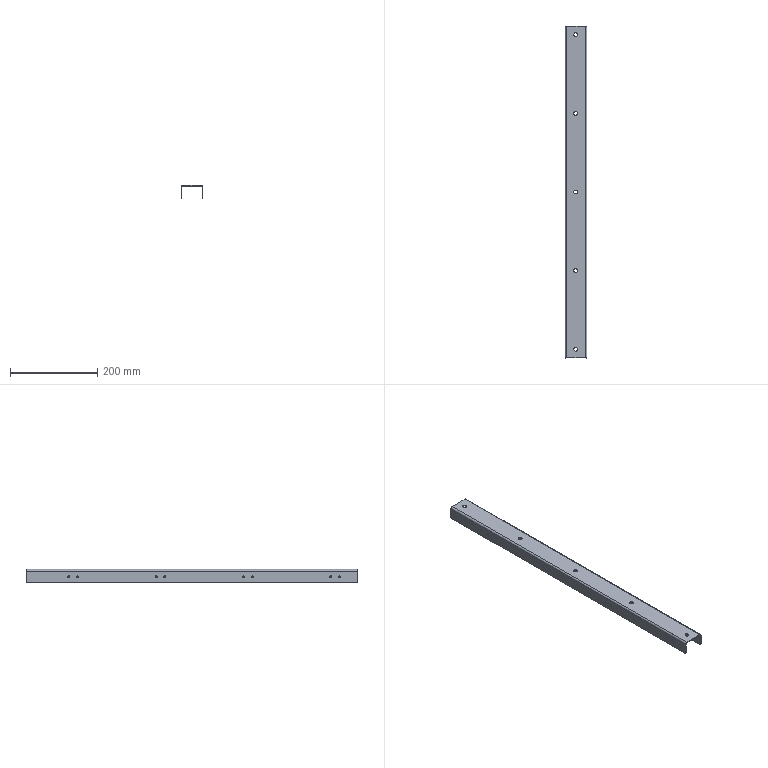Component | SolidWorks | FrameLongitudinalBeamTwo40001100-1 | 1 solid | 68 faces | volume 117929 mm3 | cylinder 50 | plane 18 | commonest cylinder face diameters 4.5 x32 9 x10 6 x4 8 x2 5 x2